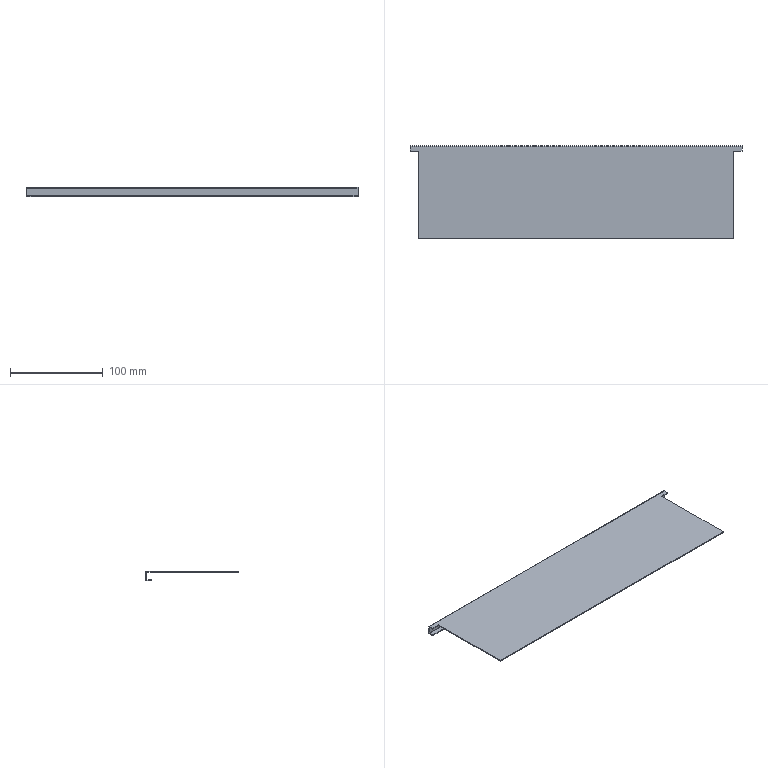Component | SolidWorks | DrawerWelding-1_DrawerBackPanel-1 | 1 solid | 30 faces | box 358 x 100 x 10 mm | volume 38932 mm3 | plane 24 | cylinder 6 | commonest cylinder face diameters 2.2 x2 0.2 x2 6 x2 | material SPCC
STEP:
#1=CARTESIAN_POINT('',(6.78,12.082,-1.529));
#2=VERTEX_POINT('',#1);
#3=CARTESIAN_POINT('',(6.544,12.082,-1.529));
#4=VERTEX_POINT('',#3);
#5=CARTESIAN_POINT('',(6.898,12.082,-1.529));
#6=DIRECTION('',(-1.,0.,0.));
#7=VECTOR('',#6,39.37);
#8=LINE('',#5,#7);
#9=EDGE_CURVE('',#2,#4,#8,.T.);
#10=ORIENTED_EDGE('',*,*,#9,.F.);
#11=CARTESIAN_POINT('',(6.78,12.082,-1.49));
#12=VERTEX_POINT('',#11);
#13=CARTESIAN_POINT('',(6.78,12.082,-1.529));
#14=DIRECTION('',(0.,0.,1.));
#15=VECTOR('',#14,39.37);
#16=LINE('',#13,#15);
#17=EDGE_CURVE('',#2,#12,#16,.T.);
#18=ORIENTED_EDGE('',*,*,#17,.T.);
#19=CARTESIAN_POINT('',(6.544,12.082,-1.49));
#20=VERTEX_POINT('',#19);
#21=CARTESIAN_POINT('',(6.898,12.082,-1.49));
#22=DIRECTION('',(-1.,0.,0.));
#23=VECTOR('',#22,39.37);
#24=LINE('',#21,#23);
#25=EDGE_CURVE('',#12,#20,#24,.T.);
#26=ORIENTED_EDGE('',*,*,#25,.T.);
#27=CARTESIAN_POINT('',(6.544,12.082,-1.529));
#28=DIRECTION('',(0.,0.,-1.));
#29=VECTOR('',#28,39.37);
#30=LINE('',#27,#29);
#31=EDGE_CURVE('',#20,#4,#30,.T.);
#32=ORIENTED_EDGE('',*,*,#31,.T.);
#33=EDGE_LOOP('',(#10,#18,#26,#32));
#34=FACE_OUTER_BOUND('',#33,.T.);
#35=CARTESIAN_POINT('',(6.898,12.082,-1.529));
#36=DIRECTION('',(0.,-1.,0.));
#37=DIRECTION('',(0.,0.,-1.));
#38=AXIS2_PLACEMENT_3D('',#35,#36,#37);
#39=PLANE('',#38);
#40=ADVANCED_FACE('',(#34),#39,.T.);
#41=CARTESIAN_POINT('',(-6.842,12.082,-1.49));
#42=VERTEX_POINT('',#41);
#43=CARTESIAN_POINT('',(-7.078,12.082,-1.49));
#44=VERTEX_POINT('',#43);
#45=CARTESIAN_POINT('',(6.898,12.082,-1.49));
#46=DIRECTION('',(-1.,0.,0.));
#47=VECTOR('',#46,39.37);
#48=LINE('',#45,#47);
#49=EDGE_CURVE('',#42,#44,#48,.T.);
#50=ORIENTED_EDGE('',*,*,#49,.T.);
#51=CARTESIAN_POINT('',(-7.078,12.082,-1.529));
#52=VERTEX_POINT('',#51);
#53=CARTESIAN_POINT('',(-7.078,12.082,-1.529));
#54=DIRECTION('',(0.,0.,-1.));
#55=VECTOR('',#54,39.37);
#56=LINE('',#53,#55);
#57=EDGE_CURVE('',#44,#52,#56,.T.);
#58=ORIENTED_EDGE('',*,*,#57,.T.);
#59=CARTESIAN_POINT('',(-6.842,12.082,-1.529));
#60=VERTEX_POINT('',#59);
#61=CARTESIAN_POINT('',(6.898,12.082,-1.529));
#62=DIRECTION('',(-1.,0.,0.));
#63=VECTOR('',#62,39.37);
#64=LINE('',#61,#63);
#65=EDGE_CURVE('',#60,#52,#64,.T.);
#66=ORIENTED_EDGE('',*,*,#65,.F.);
#67=CARTESIAN_POINT('',(-6.842,12.082,-1.529));
#68=DIRECTION('',(0.,0.,1.));
#69=VECTOR('',#68,39.37);
#70=LINE('',#67,#69);
#71=EDGE_CURVE('',#60,#42,#70,.T.);
#72=ORIENTED_EDGE('',*,*,#71,.T.);
#73=EDGE_LOOP('',(#50,#58,#66,#72));
#74=FACE_OUTER_BOUND('',#73,.T.);
#75=CARTESIAN_POINT('',(6.898,12.082,-1.529));
#76=DIRECTION('',(0.,-1.,0.));
#77=DIRECTION('',(0.,0.,-1.));
#78=AXIS2_PLACEMENT_3D('',#75,#76,#77);
#79=PLANE('',#78);
#80=ADVANCED_FACE('',(#74),#79,.T.);
#81=CARTESIAN_POINT('',(6.898,12.318,-1.179));
#82=VERTEX_POINT('',#81);
#83=CARTESIAN_POINT('',(6.898,12.278,-1.179));
#84=VERTEX_POINT('',#83);
#85=CARTESIAN_POINT('',(6.898,12.318,-1.179));
#86=DIRECTION('',(0.,-1.,-0.));
#87=VECTOR('',#86,39.37);
#88=LINE('',#85,#87);
#89=EDGE_CURVE('',#82,#84,#88,.T.);
#90=ORIENTED_EDGE('',*,*,#89,.F.);
#91=CARTESIAN_POINT('',(6.898,12.274,-1.136));
#92=VERTEX_POINT('',#91);
#93=CARTESIAN_POINT('',(6.898,12.274,-1.179));
#94=DIRECTION('',(-1.,0.,0.));
#95=DIRECTION('',(0.,0.,-1.));
#96=AXIS2_PLACEMENT_3D('',#93,#94,#95);
#97=CIRCLE('',#96,0.04331);
#98=EDGE_CURVE('',#92,#82,#97,.T.);
#99=ORIENTED_EDGE('',*,*,#98,.F.);
#100=CARTESIAN_POINT('',(6.898,12.274,-1.175));
#101=VERTEX_POINT('',#100);
#102=CARTESIAN_POINT('',(6.898,12.274,-1.175));
#103=DIRECTION('',(0.,0.,1.));
#104=VECTOR('',#103,39.37);
#105=LINE('',#102,#104);
#106=EDGE_CURVE('',#101,#92,#105,.T.);
#107=ORIENTED_EDGE('',*,*,#106,.F.);
#108=CARTESIAN_POINT('',(6.898,12.274,-1.179));
#109=DIRECTION('',(-1.,0.,0.));
#110=DIRECTION('',(0.,0.,-1.));
#111=AXIS2_PLACEMENT_3D('',#108,#109,#110);
#112=CIRCLE('',#111,0.003937);
#113=EDGE_CURVE('',#101,#84,#112,.T.);
#114=ORIENTED_EDGE('',*,*,#113,.T.);
#115=EDGE_LOOP('',(#90,#99,#107,#114));
#116=FACE_OUTER_BOUND('',#115,.T.);
#117=CARTESIAN_POINT('',(6.898,12.318,-1.179));
#118=DIRECTION('',(1.,0.,0.));
#119=DIRECTION('',(0.,0.,-1.));
#120=AXIS2_PLACEMENT_3D('',#117,#118,#119);
#121=PLANE('',#120);
#122=ADVANCED_FACE('',(#116),#121,.T.);
#123=CARTESIAN_POINT('',(6.898,12.318,-1.486));
#124=VERTEX_POINT('',#123);
#125=CARTESIAN_POINT('',(6.898,12.318,-1.136));
#126=DIRECTION('',(0.,0.,-1.));
#127=VECTOR('',#126,39.37);
#128=LINE('',#125,#127);
#129=EDGE_CURVE('',#82,#124,#128,.T.);
#130=ORIENTED_EDGE('',*,*,#129,.F.);
#131=ORIENTED_EDGE('',*,*,#89,.T.);
#132=CARTESIAN_POINT('',(6.898,12.278,-1.486));
#133=VERTEX_POINT('',#132);
#134=CARTESIAN_POINT('',(6.898,12.278,-1.136));
#135=DIRECTION('',(0.,0.,-1.));
#136=VECTOR('',#135,39.37);
#137=LINE('',#134,#136);
#138=EDGE_CURVE('',#84,#133,#137,.T.);
#139=ORIENTED_EDGE('',*,*,#138,.T.);
#140=CARTESIAN_POINT('',(6.898,12.278,-1.486));
#141=DIRECTION('',(0.,1.,0.));
#142=VECTOR('',#141,39.37);
#143=LINE('',#140,#142);
#144=EDGE_CURVE('',#133,#124,#143,.T.);
#145=ORIENTED_EDGE('',*,*,#144,.T.);
#146=EDGE_LOOP('',(#130,#131,#139,#145));
#147=FACE_OUTER_BOUND('',#146,.T.);
#148=CARTESIAN_POINT('',(6.898,12.274,-1.175));
#149=DIRECTION('',(1.,0.,0.));
#150=DIRECTION('',(0.,0.,-1.));
#151=AXIS2_PLACEMENT_3D('',#148,#149,#150);
#152=PLANE('',#151);
#153=ADVANCED_FACE('',(#147),#152,.T.);
#154=CARTESIAN_POINT('',(-7.196,12.274,-1.136));
#155=VERTEX_POINT('',#154);
#156=CARTESIAN_POINT('',(-7.196,12.274,-1.175));
#157=VERTEX_POINT('',#156);
#158=CARTESIAN_POINT('',(-7.196,12.274,-1.136));
#159=DIRECTION('',(0.,0.,-1.));
#160=VECTOR('',#159,39.37);
#161=LINE('',#158,#160);
#162=EDGE_CURVE('',#155,#157,#161,.T.);
#163=ORIENTED_EDGE('',*,*,#162,.F.);
#164=CARTESIAN_POINT('',(-7.196,12.318,-1.179));
#165=VERTEX_POINT('',#164);
#166=CARTESIAN_POINT('',(-7.196,12.274,-1.179));
#167=DIRECTION('',(-1.,0.,0.));
#168=DIRECTION('',(0.,0.,-1.));
#169=AXIS2_PLACEMENT_3D('',#166,#167,#168);
#170=CIRCLE('',#169,0.04331);
#171=EDGE_CURVE('',#155,#165,#170,.T.);
#172=ORIENTED_EDGE('',*,*,#171,.T.);
#173=CARTESIAN_POINT('',(-7.196,12.278,-1.179));
#174=VERTEX_POINT('',#173);
#175=CARTESIAN_POINT('',(-7.196,12.278,-1.179));
#176=DIRECTION('',(0.,1.,0.));
#177=VECTOR('',#176,39.37);
#178=LINE('',#175,#177);
#179=EDGE_CURVE('',#174,#165,#178,.T.);
#180=ORIENTED_EDGE('',*,*,#179,.F.);
#181=CARTESIAN_POINT('',(-7.196,12.274,-1.179));
#182=DIRECTION('',(-1.,0.,0.));
#183=DIRECTION('',(0.,0.,-1.));
#184=AXIS2_PLACEMENT_3D('',#181,#182,#183);
#185=CIRCLE('',#184,0.003937);
#186=EDGE_CURVE('',#157,#174,#185,.T.);
#187=ORIENTED_EDGE('',*,*,#186,.F.);
#188=EDGE_LOOP('',(#163,#172,#180,#187));
#189=FACE_OUTER_BOUND('',#188,.T.);
#190=CARTESIAN_POINT('',(-7.196,12.274,-1.136));
#191=DIRECTION('',(-1.,0.,0.));
#192=DIRECTION('',(0.,0.,1.));
#193=AXIS2_PLACEMENT_3D('',#190,#191,#192);
#194=PLANE('',#193);
#195=ADVANCED_FACE('',(#189),#194,.T.);
#196=CARTESIAN_POINT('',(-7.196,12.082,-1.175));
#197=VERTEX_POINT('',#196);
#198=CARTESIAN_POINT('',(-7.196,12.082,-1.136));
#199=VERTEX_POINT('',#198);
#200=CARTESIAN_POINT('',(-7.196,12.082,-1.529));
#201=DIRECTION('',(0.,0.,1.));
#202=VECTOR('',#201,39.37);
#203=LINE('',#200,#202);
#204=EDGE_CURVE('',#197,#199,#203,.T.);
#205=ORIENTED_EDGE('',*,*,#204,.T.);
#206=CARTESIAN_POINT('',(-7.196,8.381,-1.136));
#207=DIRECTION('',(0.,1.,0.));
#208=VECTOR('',#207,39.37);
#209=LINE('',#206,#208);
#210=EDGE_CURVE('',#199,#155,#209,.T.);
#211=ORIENTED_EDGE('',*,*,#210,.T.);
#212=ORIENTED_EDGE('',*,*,#162,.T.);
#213=CARTESIAN_POINT('',(-7.196,8.381,-1.175));
#214=DIRECTION('',(0.,1.,0.));
#215=VECTOR('',#214,39.37);
#216=LINE('',#213,#215);
#217=EDGE_CURVE('',#197,#157,#216,.T.);
#218=ORIENTED_EDGE('',*,*,#217,.F.);
#219=EDGE_LOOP('',(#205,#211,#212,#218));
#220=FACE_OUTER_BOUND('',#219,.T.);
#221=CARTESIAN_POINT('',(-7.196,12.278,-1.179));
#222=DIRECTION('',(-1.,0.,0.));
#223=DIRECTION('',(0.,0.,1.));
#224=AXIS2_PLACEMENT_3D('',#221,#222,#223);
#225=PLANE('',#224);
#226=ADVANCED_FACE('',(#220),#225,.T.);
#227=CARTESIAN_POINT('',(6.898,12.274,-1.529));
#228=VERTEX_POINT('',#227);
#229=CARTESIAN_POINT('',(6.898,12.274,-1.49));
#230=VERTEX_POINT('',#229);
#231=CARTESIAN_POINT('',(6.898,12.274,-1.529));
#232=DIRECTION('',(0.,0.,1.));
#233=VECTOR('',#232,39.37);
#234=LINE('',#231,#233);
#235=EDGE_CURVE('',#228,#230,#234,.T.);
#236=ORIENTED_EDGE('',*,*,#235,.F.);
#237=CARTESIAN_POINT('',(6.898,12.274,-1.486));
#238=DIRECTION('',(-1.,0.,0.));
#239=DIRECTION('',(0.,0.,-1.));
#240=AXIS2_PLACEMENT_3D('',#237,#238,#239);
#241=CIRCLE('',#240,0.04331);
#242=EDGE_CURVE('',#124,#228,#241,.T.);
#243=ORIENTED_EDGE('',*,*,#242,.F.);
#244=ORIENTED_EDGE('',*,*,#144,.F.);
#245=CARTESIAN_POINT('',(6.898,12.274,-1.486));
#246=DIRECTION('',(-1.,0.,0.));
#247=DIRECTION('',(0.,0.,-1.));
#248=AXIS2_PLACEMENT_3D('',#245,#246,#247);
#249=CIRCLE('',#248,0.003937);
#250=EDGE_CURVE('',#133,#230,#249,.T.);
#251=ORIENTED_EDGE('',*,*,#250,.T.);
#252=EDGE_LOOP('',(#236,#243,#244,#251));
#253=FACE_OUTER_BOUND('',#252,.T.);
#254=CARTESIAN_POINT('',(6.898,12.274,-1.529));
#255=DIRECTION('',(1.,0.,0.));
#256=DIRECTION('',(0.,0.,-1.));
#257=AXIS2_PLACEMENT_3D('',#254,#255,#256);
#258=PLANE('',#257);
#259=ADVANCED_FACE('',(#253),#258,.T.);
#260=CARTESIAN_POINT('',(6.898,12.2,-1.49));
#261=VERTEX_POINT('',#260);
#262=CARTESIAN_POINT('',(6.898,12.318,-1.49));
#263=DIRECTION('',(0.,-1.,0.));
#264=VECTOR('',#263,39.37);
#265=LINE('',#262,#264);
#266=EDGE_CURVE('',#230,#261,#265,.T.);
#267=ORIENTED_EDGE('',*,*,#266,.T.);
#268=CARTESIAN_POINT('',(6.898,12.2,-1.529));
#269=VERTEX_POINT('',#268);
#270=CARTESIAN_POINT('',(6.898,12.2,-1.486));
#271=DIRECTION('',(0.,0.,-1.));
#272=VECTOR('',#271,39.37);
#273=LINE('',#270,#272);
#274=EDGE_CURVE('',#261,#269,#273,.T.);
#275=ORIENTED_EDGE('',*,*,#274,.T.);
#276=CARTESIAN_POINT('',(6.898,12.318,-1.529));
#277=DIRECTION('',(0.,-1.,0.));
#278=VECTOR('',#277,39.37);
#279=LINE('',#276,#278);
#280=EDGE_CURVE('',#228,#269,#279,.T.);
#281=ORIENTED_EDGE('',*,*,#280,.F.);
#282=ORIENTED_EDGE('',*,*,#235,.T.);
#283=EDGE_LOOP('',(#267,#275,#281,#282));
#284=FACE_OUTER_BOUND('',#283,.T.);
#285=CARTESIAN_POINT('',(6.898,12.278,-1.486));
#286=DIRECTION('',(1.,0.,0.));
#287=DIRECTION('',(0.,0.,-1.));
#288=AXIS2_PLACEMENT_3D('',#285,#286,#287);
#289=PLANE('',#288);
#290=ADVANCED_FACE('',(#284),#289,.T.);
#291=CARTESIAN_POINT('',(-7.196,12.318,-1.486));
#292=VERTEX_POINT('',#291);
#293=CARTESIAN_POINT('',(-7.196,12.278,-1.486));
#294=VERTEX_POINT('',#293);
#295=CARTESIAN_POINT('',(-7.196,12.318,-1.486));
#296=DIRECTION('',(0.,-1.,-0.));
#297=VECTOR('',#296,39.37);
#298=LINE('',#295,#297);
#299=EDGE_CURVE('',#292,#294,#298,.T.);
#300=ORIENTED_EDGE('',*,*,#299,.F.);
#301=CARTESIAN_POINT('',(-7.196,12.274,-1.529));
#302=VERTEX_POINT('',#301);
#303=CARTESIAN_POINT('',(-7.196,12.274,-1.486));
#304=DIRECTION('',(-1.,0.,0.));
#305=DIRECTION('',(0.,0.,-1.));
#306=AXIS2_PLACEMENT_3D('',#303,#304,#305);
#307=CIRCLE('',#306,0.04331);
#308=EDGE_CURVE('',#292,#302,#307,.T.);
#309=ORIENTED_EDGE('',*,*,#308,.T.);
#310=CARTESIAN_POINT('',(-7.196,12.274,-1.49));
#311=VERTEX_POINT('',#310);
#312=CARTESIAN_POINT('',(-7.196,12.274,-1.49));
#313=DIRECTION('',(0.,0.,-1.));
#314=VECTOR('',#313,39.37);
#315=LINE('',#312,#314);
#316=EDGE_CURVE('',#311,#302,#315,.T.);
#317=ORIENTED_EDGE('',*,*,#316,.F.);
#318=CARTESIAN_POINT('',(-7.196,12.274,-1.486));
#319=DIRECTION('',(-1.,0.,0.));
#320=DIRECTION('',(0.,0.,-1.));
#321=AXIS2_PLACEMENT_3D('',#318,#319,#320);
#322=CIRCLE('',#321,0.003937);
#323=EDGE_CURVE('',#294,#311,#322,.T.);
#324=ORIENTED_EDGE('',*,*,#323,.F.);
#325=EDGE_LOOP('',(#300,#309,#317,#324));
#326=FACE_OUTER_BOUND('',#325,.T.);
#327=CARTESIAN_POINT('',(-7.196,12.318,-1.486));
#328=DIRECTION('',(-1.,0.,0.));
#329=DIRECTION('',(0.,0.,1.));
#330=AXIS2_PLACEMENT_3D('',#327,#328,#329);
#331=PLANE('',#330);
#332=ADVANCED_FACE('',(#326),#331,.T.);
#333=CARTESIAN_POINT('',(-7.196,12.318,-1.136));
#334=DIRECTION('',(0.,0.,-1.));
#335=VECTOR('',#334,39.37);
#336=LINE('',#333,#335);
#337=EDGE_CURVE('',#165,#292,#336,.T.);
#338=ORIENTED_EDGE('',*,*,#337,.T.);
#339=ORIENTED_EDGE('',*,*,#299,.T.);
#340=CARTESIAN_POINT('',(-7.196,12.278,-1.136));
#341=DIRECTION('',(0.,0.,-1.));
#342=VECTOR('',#341,39.37);
#343=LINE('',#340,#342);
#344=EDGE_CURVE('',#174,#294,#343,.T.);
#345=ORIENTED_EDGE('',*,*,#344,.F.);
#346=ORIENTED_EDGE('',*,*,#179,.T.);
#347=EDGE_LOOP('',(#338,#339,#345,#346));
#348=FACE_OUTER_BOUND('',#347,.T.);
#349=CARTESIAN_POINT('',(-7.196,12.274,-1.49));
#350=DIRECTION('',(-1.,0.,0.));
#351=DIRECTION('',(0.,0.,1.));
#352=AXIS2_PLACEMENT_3D('',#349,#350,#351);
#353=PLANE('',#352);
#354=ADVANCED_FACE('',(#348),#353,.T.);
#355=ORIENTED_EDGE('',*,*,#25,.F.);
#356=CARTESIAN_POINT('',(6.78,12.2,-1.49));
#357=DIRECTION('',(0.,0.,1.));
#358=DIRECTION('',(-1.,0.,0.));
#359=AXIS2_PLACEMENT_3D('',#356,#357,#358);
#360=CIRCLE('',#359,0.1181);
#361=EDGE_CURVE('',#12,#261,#360,.T.);
#362=ORIENTED_EDGE('',*,*,#361,.T.);
#363=ORIENTED_EDGE('',*,*,#266,.F.);
#364=CARTESIAN_POINT('',(6.898,12.274,-1.49));
#365=DIRECTION('',(-1.,0.,0.));
#366=VECTOR('',#365,39.37);
#367=LINE('',#364,#366);
#368=EDGE_CURVE('',#230,#311,#367,.T.);
#369=ORIENTED_EDGE('',*,*,#368,.T.);
#370=CARTESIAN_POINT('',(-7.196,12.2,-1.49));
#371=VERTEX_POINT('',#370);
#372=CARTESIAN_POINT('',(-7.196,12.318,-1.49));
#373=DIRECTION('',(0.,-1.,0.));
#374=VECTOR('',#373,39.37);
#375=LINE('',#372,#374);
#376=EDGE_CURVE('',#311,#371,#375,.T.);
#377=ORIENTED_EDGE('',*,*,#376,.T.);
#378=CARTESIAN_POINT('',(-7.078,12.2,-1.49));
#379=DIRECTION('',(0.,0.,1.));
#380=DIRECTION('',(-1.,0.,0.));
#381=AXIS2_PLACEMENT_3D('',#378,#379,#380);
#382=CIRCLE('',#381,0.1181);
#383=EDGE_CURVE('',#371,#44,#382,.T.);
#384=ORIENTED_EDGE('',*,*,#383,.T.);
#385=ORIENTED_EDGE('',*,*,#49,.F.);
#386=CARTESIAN_POINT('',(6.898,12.082,-1.49));
#387=DIRECTION('',(-1.,0.,0.));
#388=VECTOR('',#387,39.37);
#389=LINE('',#386,#388);
#390=EDGE_CURVE('',#20,#42,#389,.T.);
#391=ORIENTED_EDGE('',*,*,#390,.F.);
#392=EDGE_LOOP('',(#355,#362,#363,#369,#377,#384,#385,#391));
#393=FACE_OUTER_BOUND('',#392,.T.);
#394=CARTESIAN_POINT('',(6.898,12.318,-1.49));
#395=DIRECTION('',(0.,0.,-1.));
#396=DIRECTION('',(-1.,0.,0.));
#397=AXIS2_PLACEMENT_3D('',#394,#395,#396);
#398=PLANE('',#397);
#399=ADVANCED_FACE('',(#393),#398,.F.);
#400=ORIENTED_EDGE('',*,*,#31,.F.);
#401=ORIENTED_EDGE('',*,*,#390,.T.);
#402=ORIENTED_EDGE('',*,*,#71,.F.);
#403=CARTESIAN_POINT('',(6.898,12.082,-1.529));
#404=DIRECTION('',(-1.,0.,0.));
#405=VECTOR('',#404,39.37);
#406=LINE('',#403,#405);
#407=EDGE_CURVE('',#4,#60,#406,.T.);
#408=ORIENTED_EDGE('',*,*,#407,.F.);
#409=EDGE_LOOP('',(#400,#401,#402,#408));
#410=FACE_OUTER_BOUND('',#409,.T.);
#411=CARTESIAN_POINT('',(6.898,12.082,-1.529));
#412=DIRECTION('',(0.,-1.,0.));
#413=DIRECTION('',(0.,0.,-1.));
#414=AXIS2_PLACEMENT_3D('',#411,#412,#413);
#415=PLANE('',#414);
#416=ADVANCED_FACE('',(#410),#415,.T.);
#417=ORIENTED_EDGE('',*,*,#280,.T.);
#418=CARTESIAN_POINT('',(6.78,12.2,-1.529));
#419=DIRECTION('',(0.,0.,-1.));
#420=DIRECTION('',(-1.,0.,0.));
#421=AXIS2_PLACEMENT_3D('',#418,#419,#420);
#422=CIRCLE('',#421,0.1181);
#423=EDGE_CURVE('',#269,#2,#422,.T.);
#424=ORIENTED_EDGE('',*,*,#423,.T.);
#425=ORIENTED_EDGE('',*,*,#9,.T.);
#426=ORIENTED_EDGE('',*,*,#407,.T.);
#427=ORIENTED_EDGE('',*,*,#65,.T.);
#428=CARTESIAN_POINT('',(-7.196,12.2,-1.529));
#429=VERTEX_POINT('',#428);
#430=CARTESIAN_POINT('',(-7.078,12.2,-1.529));
#431=DIRECTION('',(0.,0.,-1.));
#432=DIRECTION('',(-1.,0.,0.));
#433=AXIS2_PLACEMENT_3D('',#430,#431,#432);
#434=CIRCLE('',#433,0.1181);
#435=EDGE_CURVE('',#52,#429,#434,.T.);
#436=ORIENTED_EDGE('',*,*,#435,.T.);
#437=CARTESIAN_POINT('',(-7.196,12.318,-1.529));
#438=DIRECTION('',(0.,-1.,0.));
#439=VECTOR('',#438,39.37);
#440=LINE('',#437,#439);
#441=EDGE_CURVE('',#302,#429,#440,.T.);
#442=ORIENTED_EDGE('',*,*,#441,.F.);
#443=CARTESIAN_POINT('',(6.898,12.274,-1.529));
#444=DIRECTION('',(-1.,0.,0.));
#445=VECTOR('',#444,39.37);
#446=LINE('',#443,#445);
#447=EDGE_CURVE('',#228,#302,#446,.T.);
#448=ORIENTED_EDGE('',*,*,#447,.F.);
#449=EDGE_LOOP('',(#417,#424,#425,#426,#427,#436,#442,#448));
#450=FACE_OUTER_BOUND('',#449,.T.);
#451=CARTESIAN_POINT('',(6.898,12.318,-1.529));
#452=DIRECTION('',(0.,0.,-1.));
#453=DIRECTION('',(-1.,0.,0.));
#454=AXIS2_PLACEMENT_3D('',#451,#452,#453);
#455=PLANE('',#454);
#456=ADVANCED_FACE('',(#450),#455,.T.);
#457=ORIENTED_EDGE('',*,*,#308,.F.);
#458=CARTESIAN_POINT('',(6.898,12.318,-1.486));
#459=DIRECTION('',(-1.,0.,0.));
#460=VECTOR('',#459,39.37);
#461=LINE('',#458,#460);
#462=EDGE_CURVE('',#124,#292,#461,.T.);
#463=ORIENTED_EDGE('',*,*,#462,.F.);
#464=ORIENTED_EDGE('',*,*,#242,.T.);
#465=ORIENTED_EDGE('',*,*,#447,.T.);
#466=EDGE_LOOP('',(#457,#463,#464,#465));
#467=FACE_OUTER_BOUND('',#466,.T.);
#468=CARTESIAN_POINT('',(6.898,12.274,-1.486));
#469=DIRECTION('',(-1.,0.,0.));
#470=DIRECTION('',(0.,0.,1.));
#471=AXIS2_PLACEMENT_3D('',#468,#469,#470);
#472=CYLINDRICAL_SURFACE('',#471,0.04331);
#473=ADVANCED_FACE('',(#467),#472,.T.);
#474=ORIENTED_EDGE('',*,*,#337,.F.);
#475=CARTESIAN_POINT('',(6.898,12.318,-1.179));
#476=DIRECTION('',(-1.,0.,0.));
#477=VECTOR('',#476,39.37);
#478=LINE('',#475,#477);
#479=EDGE_CURVE('',#82,#165,#478,.T.);
#480=ORIENTED_EDGE('',*,*,#479,.F.);
#481=ORIENTED_EDGE('',*,*,#129,.T.);
#482=ORIENTED_EDGE('',*,*,#462,.T.);
#483=EDGE_LOOP('',(#474,#480,#481,#482));
#484=FACE_OUTER_BOUND('',#483,.T.);
#485=CARTESIAN_POINT('',(6.898,12.318,-1.136));
#486=DIRECTION('',(0.,1.,0.));
#487=DIRECTION('',(0.,-0.,1.));
#488=AXIS2_PLACEMENT_3D('',#485,#486,#487);
#489=PLANE('',#488);
#490=ADVANCED_FACE('',(#484),#489,.T.);
#491=ORIENTED_EDGE('',*,*,#171,.F.);
#492=CARTESIAN_POINT('',(6.898,12.274,-1.136));
#493=DIRECTION('',(-1.,0.,0.));
#494=VECTOR('',#493,39.37);
#495=LINE('',#492,#494);
#496=EDGE_CURVE('',#92,#155,#495,.T.);
#497=ORIENTED_EDGE('',*,*,#496,.F.);
#498=ORIENTED_EDGE('',*,*,#98,.T.);
#499=ORIENTED_EDGE('',*,*,#479,.T.);
#500=EDGE_LOOP('',(#491,#497,#498,#499));
#501=FACE_OUTER_BOUND('',#500,.T.);
#502=CARTESIAN_POINT('',(6.898,12.274,-1.179));
#503=DIRECTION('',(-1.,0.,0.));
#504=DIRECTION('',(0.,0.,1.));
#505=AXIS2_PLACEMENT_3D('',#502,#503,#504);
#506=CYLINDRICAL_SURFACE('',#505,0.04331);
#507=ADVANCED_FACE('',(#501),#506,.T.);
#508=CARTESIAN_POINT('',(6.544,12.082,-1.136));
#509=VERTEX_POINT('',#508);
#510=CARTESIAN_POINT('',(6.544,8.381,-1.136));
#511=VERTEX_POINT('',#510);
#512=CARTESIAN_POINT('',(6.544,8.381,-1.136));
#513=DIRECTION('',(0.,-1.,0.));
#514=VECTOR('',#513,39.37);
#515=LINE('',#512,#514);
#516=EDGE_CURVE('',#509,#511,#515,.T.);
#517=ORIENTED_EDGE('',*,*,#516,.F.);
#518=CARTESIAN_POINT('',(6.898,12.082,-1.136));
#519=VERTEX_POINT('',#518);
#520=CARTESIAN_POINT('',(6.898,12.082,-1.136));
#521=DIRECTION('',(-1.,0.,0.));
#522=VECTOR('',#521,39.37);
#523=LINE('',#520,#522);
#524=EDGE_CURVE('',#519,#509,#523,.T.);
#525=ORIENTED_EDGE('',*,*,#524,.F.);
#526=CARTESIAN_POINT('',(6.898,8.381,-1.136));
#527=DIRECTION('',(0.,1.,0.));
#528=VECTOR('',#527,39.37);
#529=LINE('',#526,#528);
#530=EDGE_CURVE('',#519,#92,#529,.T.);
#531=ORIENTED_EDGE('',*,*,#530,.T.);
#532=ORIENTED_EDGE('',*,*,#496,.T.);
#533=ORIENTED_EDGE('',*,*,#210,.F.);
#534=CARTESIAN_POINT('',(-6.842,12.082,-1.136));
#535=VERTEX_POINT('',#534);
#536=CARTESIAN_POINT('',(-7.196,12.082,-1.136));
#537=DIRECTION('',(-1.,0.,0.));
#538=VECTOR('',#537,39.37);
#539=LINE('',#536,#538);
#540=EDGE_CURVE('',#535,#199,#539,.T.);
#541=ORIENTED_EDGE('',*,*,#540,.F.);
#542=CARTESIAN_POINT('',(-6.842,8.381,-1.136));
#543=VERTEX_POINT('',#542);
#544=CARTESIAN_POINT('',(-6.842,12.082,-1.136));
#545=DIRECTION('',(-0.,1.,0.));
#546=VECTOR('',#545,39.37);
#547=LINE('',#544,#546);
#548=EDGE_CURVE('',#543,#535,#547,.T.);
#549=ORIENTED_EDGE('',*,*,#548,.F.);
#550=CARTESIAN_POINT('',(6.898,8.381,-1.136));
#551=DIRECTION('',(-1.,0.,0.));
#552=VECTOR('',#551,39.37);
#553=LINE('',#550,#552);
#554=EDGE_CURVE('',#511,#543,#553,.T.);
#555=ORIENTED_EDGE('',*,*,#554,.F.);
#556=EDGE_LOOP('',(#517,#525,#531,#532,#533,#541,#549,#555));
#557=FACE_OUTER_BOUND('',#556,.T.);
#558=CARTESIAN_POINT('',(6.898,8.381,-1.136));
#559=DIRECTION('',(0.,0.,1.));
#560=DIRECTION('',(1.,0.,0.));
#561=AXIS2_PLACEMENT_3D('',#558,#559,#560);
#562=PLANE('',#561);
#563=ADVANCED_FACE('',(#557),#562,.T.);
#564=CARTESIAN_POINT('',(6.544,8.381,-1.175));
#565=VERTEX_POINT('',#564);
#566=CARTESIAN_POINT('',(6.544,8.381,-1.529));
#567=DIRECTION('',(0.,0.,1.));
#568=VECTOR('',#567,39.37);
#569=LINE('',#566,#568);
#570=EDGE_CURVE('',#565,#511,#569,.T.);
#571=ORIENTED_EDGE('',*,*,#570,.T.);
#572=ORIENTED_EDGE('',*,*,#554,.T.);
#573=CARTESIAN_POINT('',(-6.842,8.381,-1.175));
#574=VERTEX_POINT('',#573);
#575=CARTESIAN_POINT('',(-6.842,8.381,-1.529));
#576=DIRECTION('',(0.,0.,1.));
#577=VECTOR('',#576,39.37);
#578=LINE('',#575,#577);
#579=EDGE_CURVE('',#574,#543,#578,.T.);
#580=ORIENTED_EDGE('',*,*,#579,.F.);
#581=CARTESIAN_POINT('',(6.898,8.381,-1.175));
#582=DIRECTION('',(-1.,0.,0.));
#583=VECTOR('',#582,39.37);
#584=LINE('',#581,#583);
#585=EDGE_CURVE('',#565,#574,#584,.T.);
#586=ORIENTED_EDGE('',*,*,#585,.F.);
#587=EDGE_LOOP('',(#571,#572,#580,#586));
#588=FACE_OUTER_BOUND('',#587,.T.);
#589=CARTESIAN_POINT('',(6.898,8.381,-1.175));
#590=DIRECTION('',(0.,-1.,0.));
#591=DIRECTION('',(0.,0.,-1.));
#592=AXIS2_PLACEMENT_3D('',#589,#590,#591);
#593=PLANE('',#592);
#594=ADVANCED_FACE('',(#588),#593,.T.);
#595=CARTESIAN_POINT('',(6.898,12.082,-1.175));
#596=VERTEX_POINT('',#595);
#597=CARTESIAN_POINT('',(6.544,12.082,-1.175));
#598=VERTEX_POINT('',#597);
#599=CARTESIAN_POINT('',(6.898,12.082,-1.175));
#600=DIRECTION('',(-1.,0.,0.));
#601=VECTOR('',#600,39.37);
#602=LINE('',#599,#601);
#603=EDGE_CURVE('',#596,#598,#602,.T.);
#604=ORIENTED_EDGE('',*,*,#603,.T.);
#605=CARTESIAN_POINT('',(6.544,8.381,-1.175));
#606=DIRECTION('',(0.,-1.,0.));
#607=VECTOR('',#606,39.37);
#608=LINE('',#605,#607);
#609=EDGE_CURVE('',#598,#565,#608,.T.);
#610=ORIENTED_EDGE('',*,*,#609,.T.);
#611=ORIENTED_EDGE('',*,*,#585,.T.);
#612=CARTESIAN_POINT('',(-6.842,12.082,-1.175));
#613=VERTEX_POINT('',#612);
#614=CARTESIAN_POINT('',(-6.842,8.381,-1.175));
#615=DIRECTION('',(-0.,1.,0.));
#616=VECTOR('',#615,39.37);
#617=LINE('',#614,#616);
#618=EDGE_CURVE('',#574,#613,#617,.T.);
#619=ORIENTED_EDGE('',*,*,#618,.T.);
#620=CARTESIAN_POINT('',(6.898,12.082,-1.175));
#621=DIRECTION('',(-1.,0.,0.));
#622=VECTOR('',#621,39.37);
#623=LINE('',#620,#622);
#624=EDGE_CURVE('',#613,#197,#623,.T.);
#625=ORIENTED_EDGE('',*,*,#624,.T.);
#626=ORIENTED_EDGE('',*,*,#217,.T.);
#627=CARTESIAN_POINT('',(6.898,12.274,-1.175));
#628=DIRECTION('',(-1.,0.,0.));
#629=VECTOR('',#628,39.37);
#630=LINE('',#627,#629);
#631=EDGE_CURVE('',#101,#157,#630,.T.);
#632=ORIENTED_EDGE('',*,*,#631,.F.);
#633=CARTESIAN_POINT('',(6.898,8.381,-1.175));
#634=DIRECTION('',(0.,1.,0.));
#635=VECTOR('',#634,39.37);
#636=LINE('',#633,#635);
#637=EDGE_CURVE('',#596,#101,#636,.T.);
#638=ORIENTED_EDGE('',*,*,#637,.F.);
#639=EDGE_LOOP('',(#604,#610,#611,#619,#625,#626,#632,#638));
#640=FACE_OUTER_BOUND('',#639,.T.);
#641=CARTESIAN_POINT('',(6.898,8.381,-1.175));
#642=DIRECTION('',(0.,0.,1.));
#643=DIRECTION('',(1.,0.,0.));
#644=AXIS2_PLACEMENT_3D('',#641,#642,#643);
#645=PLANE('',#644);
#646=ADVANCED_FACE('',(#640),#645,.F.);
#647=ORIENTED_EDGE('',*,*,#186,.T.);
#648=CARTESIAN_POINT('',(6.898,12.278,-1.179));
#649=DIRECTION('',(-1.,0.,0.));
#650=VECTOR('',#649,39.37);
#651=LINE('',#648,#650);
#652=EDGE_CURVE('',#84,#174,#651,.T.);
#653=ORIENTED_EDGE('',*,*,#652,.F.);
#654=ORIENTED_EDGE('',*,*,#113,.F.);
#655=ORIENTED_EDGE('',*,*,#631,.T.);
#656=EDGE_LOOP('',(#647,#653,#654,#655));
#657=FACE_OUTER_BOUND('',#656,.T.);
#658=CARTESIAN_POINT('',(6.898,12.274,-1.179));
#659=DIRECTION('',(-1.,0.,0.));
#660=DIRECTION('',(0.,0.,1.));
#661=AXIS2_PLACEMENT_3D('',#658,#659,#660);
#662=CYLINDRICAL_SURFACE('',#661,0.003937);
#663=ADVANCED_FACE('',(#657),#662,.F.);
#664=ORIENTED_EDGE('',*,*,#344,.T.);
#665=CARTESIAN_POINT('',(6.898,12.278,-1.486));
#666=DIRECTION('',(-1.,0.,0.));
#667=VECTOR('',#666,39.37);
#668=LINE('',#665,#667);
#669=EDGE_CURVE('',#133,#294,#668,.T.);
#670=ORIENTED_EDGE('',*,*,#669,.F.);
#671=ORIENTED_EDGE('',*,*,#138,.F.);
#672=ORIENTED_EDGE('',*,*,#652,.T.);
#673=EDGE_LOOP('',(#664,#670,#671,#672));
#674=FACE_OUTER_BOUND('',#673,.T.);
#675=CARTESIAN_POINT('',(6.898,12.278,-1.136));
#676=DIRECTION('',(0.,1.,0.));
#677=DIRECTION('',(0.,-0.,1.));
#678=AXIS2_PLACEMENT_3D('',#675,#676,#677);
#679=PLANE('',#678);
#680=ADVANCED_FACE('',(#674),#679,.F.);
#681=ORIENTED_EDGE('',*,*,#323,.T.);
#682=ORIENTED_EDGE('',*,*,#368,.F.);
#683=ORIENTED_EDGE('',*,*,#250,.F.);
#684=ORIENTED_EDGE('',*,*,#669,.T.);
#685=EDGE_LOOP('',(#681,#682,#683,#684));
#686=FACE_OUTER_BOUND('',#685,.T.);
#687=CARTESIAN_POINT('',(6.898,12.274,-1.486));
#688=DIRECTION('',(-1.,0.,0.));
#689=DIRECTION('',(0.,0.,1.));
#690=AXIS2_PLACEMENT_3D('',#687,#688,#689);
#691=CYLINDRICAL_SURFACE('',#690,0.003937);
#692=ADVANCED_FACE('',(#686),#691,.F.);
#693=CARTESIAN_POINT('',(6.898,12.082,-1.486));
#694=DIRECTION('',(0.,0.,1.));
#695=VECTOR('',#694,39.37);
#696=LINE('',#693,#695);
#697=EDGE_CURVE('',#596,#519,#696,.T.);
#698=ORIENTED_EDGE('',*,*,#697,.F.);
#699=ORIENTED_EDGE('',*,*,#637,.T.);
#700=ORIENTED_EDGE('',*,*,#106,.T.);
#701=ORIENTED_EDGE('',*,*,#530,.F.);
#702=EDGE_LOOP('',(#698,#699,#700,#701));
#703=FACE_OUTER_BOUND('',#702,.T.);
#704=CARTESIAN_POINT('',(6.898,12.274,-1.486));
#705=DIRECTION('',(1.,0.,0.));
#706=DIRECTION('',(0.,0.,-1.));
#707=AXIS2_PLACEMENT_3D('',#704,#705,#706);
#708=PLANE('',#707);
#709=ADVANCED_FACE('',(#703),#708,.T.);
#710=ORIENTED_EDGE('',*,*,#441,.T.);
#711=CARTESIAN_POINT('',(-7.196,12.2,-1.49));
#712=DIRECTION('',(0.,0.,1.));
#713=VECTOR('',#712,39.37);
#714=LINE('',#711,#713);
#715=EDGE_CURVE('',#429,#371,#714,.T.);
#716=ORIENTED_EDGE('',*,*,#715,.T.);
#717=ORIENTED_EDGE('',*,*,#376,.F.);
#718=ORIENTED_EDGE('',*,*,#316,.T.);
#719=EDGE_LOOP('',(#710,#716,#717,#718));
#720=FACE_OUTER_BOUND('',#719,.T.);
#721=CARTESIAN_POINT('',(-7.196,12.274,-1.486));
#722=DIRECTION('',(1.,0.,0.));
#723=DIRECTION('',(0.,0.,-1.));
#724=AXIS2_PLACEMENT_3D('',#721,#722,#723);
#725=PLANE('',#724);
#726=ADVANCED_FACE('',(#720),#725,.F.);
#727=CARTESIAN_POINT('',(-6.842,12.082,-1.529));
#728=DIRECTION('',(0.,0.,1.));
#729=VECTOR('',#728,39.37);
#730=LINE('',#727,#729);
#731=EDGE_CURVE('',#613,#535,#730,.T.);
#732=ORIENTED_EDGE('',*,*,#731,.T.);
#733=ORIENTED_EDGE('',*,*,#540,.T.);
#734=ORIENTED_EDGE('',*,*,#204,.F.);
#735=ORIENTED_EDGE('',*,*,#624,.F.);
#736=EDGE_LOOP('',(#732,#733,#734,#735));
#737=FACE_OUTER_BOUND('',#736,.T.);
#738=CARTESIAN_POINT('',(-7.196,12.082,-1.529));
#739=DIRECTION('',(0.,1.,0.));
#740=DIRECTION('',(0.,0.,1.));
#741=AXIS2_PLACEMENT_3D('',#738,#739,#740);
#742=PLANE('',#741);
#743=ADVANCED_FACE('',(#737),#742,.F.);
#744=ORIENTED_EDGE('',*,*,#579,.T.);
#745=ORIENTED_EDGE('',*,*,#548,.T.);
#746=ORIENTED_EDGE('',*,*,#731,.F.);
#747=ORIENTED_EDGE('',*,*,#618,.F.);
#748=EDGE_LOOP('',(#744,#745,#746,#747));
#749=FACE_OUTER_BOUND('',#748,.T.);
#750=CARTESIAN_POINT('',(-6.842,12.082,-1.529));
#751=DIRECTION('',(1.,0.,0.));
#752=DIRECTION('',(-0.,1.,0.));
#753=AXIS2_PLACEMENT_3D('',#750,#751,#752);
#754=PLANE('',#753);
#755=ADVANCED_FACE('',(#749),#754,.F.);
#756=CARTESIAN_POINT('',(6.544,12.082,-1.529));
#757=DIRECTION('',(0.,0.,1.));
#758=VECTOR('',#757,39.37);
#759=LINE('',#756,#758);
#760=EDGE_CURVE('',#598,#509,#759,.T.);
#761=ORIENTED_EDGE('',*,*,#760,.T.);
#762=ORIENTED_EDGE('',*,*,#516,.T.);
#763=ORIENTED_EDGE('',*,*,#570,.F.);
#764=ORIENTED_EDGE('',*,*,#609,.F.);
#765=EDGE_LOOP('',(#761,#762,#763,#764));
#766=FACE_OUTER_BOUND('',#765,.T.);
#767=CARTESIAN_POINT('',(6.544,8.381,-1.529));
#768=DIRECTION('',(-1.,0.,0.));
#769=DIRECTION('',(0.,0.,1.));
#770=AXIS2_PLACEMENT_3D('',#767,#768,#769);
#771=PLANE('',#770);
#772=ADVANCED_FACE('',(#766),#771,.F.);
#773=ORIENTED_EDGE('',*,*,#697,.T.);
#774=ORIENTED_EDGE('',*,*,#524,.T.);
#775=ORIENTED_EDGE('',*,*,#760,.F.);
#776=ORIENTED_EDGE('',*,*,#603,.F.);
#777=EDGE_LOOP('',(#773,#774,#775,#776));
#778=FACE_OUTER_BOUND('',#777,.T.);
#779=CARTESIAN_POINT('',(6.898,12.082,-1.529));
#780=DIRECTION('',(0.,1.,0.));
#781=DIRECTION('',(0.,0.,1.));
#782=AXIS2_PLACEMENT_3D('',#779,#780,#781);
#783=PLANE('',#782);
#784=ADVANCED_FACE('',(#778),#783,.F.);
#785=ORIENTED_EDGE('',*,*,#423,.F.);
#786=ORIENTED_EDGE('',*,*,#274,.F.);
#787=ORIENTED_EDGE('',*,*,#361,.F.);
#788=ORIENTED_EDGE('',*,*,#17,.F.);
#789=EDGE_LOOP('',(#785,#786,#787,#788));
#790=FACE_OUTER_BOUND('',#789,.T.);
#791=CARTESIAN_POINT('',(6.78,12.2,-1.529));
#792=DIRECTION('',(0.,0.,1.));
#793=DIRECTION('',(1.,0.,0.));
#794=AXIS2_PLACEMENT_3D('',#791,#792,#793);
#795=CYLINDRICAL_SURFACE('',#794,0.1181);
#796=ADVANCED_FACE('',(#790),#795,.T.);
#797=ORIENTED_EDGE('',*,*,#435,.F.);
#798=ORIENTED_EDGE('',*,*,#57,.F.);
#799=ORIENTED_EDGE('',*,*,#383,.F.);
#800=ORIENTED_EDGE('',*,*,#715,.F.);
#801=EDGE_LOOP('',(#797,#798,#799,#800));
#802=FACE_OUTER_BOUND('',#801,.T.);
#803=CARTESIAN_POINT('',(-7.078,12.2,-1.486));
#804=DIRECTION('',(0.,0.,-1.));
#805=DIRECTION('',(-1.,0.,0.));
#806=AXIS2_PLACEMENT_3D('',#803,#804,#805);
#807=CYLINDRICAL_SURFACE('',#806,0.1181);
#808=ADVANCED_FACE('',(#802),#807,.T.);
#809=CLOSED_SHELL('',(#40,#80,#122,#153,#195,#226,#259,#290,#332,#354,#399,#416,#456,#473,#490,#507,#563,#594,#646,#663,#680,#692,#709,#726,#743,#755,#772,#784,#796,#808));
#810=MANIFOLD_SOLID_BREP('',#809);
#811=CARTESIAN_POINT('',(0.,0.,0.));
#812=DIRECTION('',(0.,0.,1.));
#813=DIRECTION('',(1.,0.,0.));
#814=AXIS2_PLACEMENT_3D('',#811,#812,#813);
#815=(LENGTH_UNIT()NAMED_UNIT(*)SI_UNIT($,.METRE.));
#816=LENGTH_MEASURE_WITH_UNIT(LENGTH_MEASURE(0.0254),#815);
#817=DIMENSIONAL_EXPONENTS(1.,0.,0.,0.,0.,0.,0.);
#818=(CONVERSION_BASED_UNIT('',#816)LENGTH_UNIT()NAMED_UNIT(#817));
#819=UNCERTAINTY_MEASURE_WITH_UNIT(LENGTH_MEASURE(0.00001),#818,'','');
#820=(NAMED_UNIT(*)PLANE_ANGLE_UNIT()SI_UNIT($,.RADIAN.));
#821=(NAMED_UNIT(*)SI_UNIT($,.STERADIAN.)SOLID_ANGLE_UNIT());
#822=(GEOMETRIC_REPRESENTATION_CONTEXT(3)GLOBAL_UNCERTAINTY_ASSIGNED_CONTEXT((#819))GLOBAL_UNIT_ASSIGNED_CONTEXT((#818,#820,#821))REPRESENTATION_CONTEXT('',''));
#823=ADVANCED_BREP_SHAPE_REPRESENTATION('',(#810,#814),#822);
#824=COLOUR_RGB('',0.7922,0.8196,0.9333);
#825=FILL_AREA_STYLE_COLOUR('',#824);
#826=FILL_AREA_STYLE('',(#825));
#827=SURFACE_STYLE_FILL_AREA(#826);
#828=SURFACE_SIDE_STYLE('',(#827));
#829=SURFACE_STYLE_USAGE(.BOTH.,#828);
#830=PRESENTATION_STYLE_ASSIGNMENT((#829));
#831=STYLED_ITEM('',(#830),#810);
#832=(LENGTH_UNIT()NAMED_UNIT(*)SI_UNIT($,.METRE.));
#833=LENGTH_MEASURE_WITH_UNIT(LENGTH_MEASURE(0.0254),#832);
#834=DIMENSIONAL_EXPONENTS(1.,0.,0.,0.,0.,0.,0.);
#835=(CONVERSION_BASED_UNIT('',#833)LENGTH_UNIT()NAMED_UNIT(#834));
#836=UNCERTAINTY_MEASURE_WITH_UNIT(LENGTH_MEASURE(0.00001),#835,'','');
#837=(NAMED_UNIT(*)PLANE_ANGLE_UNIT()SI_UNIT($,.RADIAN.));
#838=(NAMED_UNIT(*)SI_UNIT($,.STERADIAN.)SOLID_ANGLE_UNIT());
#839=(GEOMETRIC_REPRESENTATION_CONTEXT(3)GLOBAL_UNCERTAINTY_ASSIGNED_CONTEXT((#836))GLOBAL_UNIT_ASSIGNED_CONTEXT((#835,#837,#838))REPRESENTATION_CONTEXT('',''));
#840=MECHANICAL_DESIGN_GEOMETRIC_PRESENTATION_REPRESENTATION('',(#831),#839);
#841=PRESENTATION_LAYER_ASSIGNMENT('','',(#831));